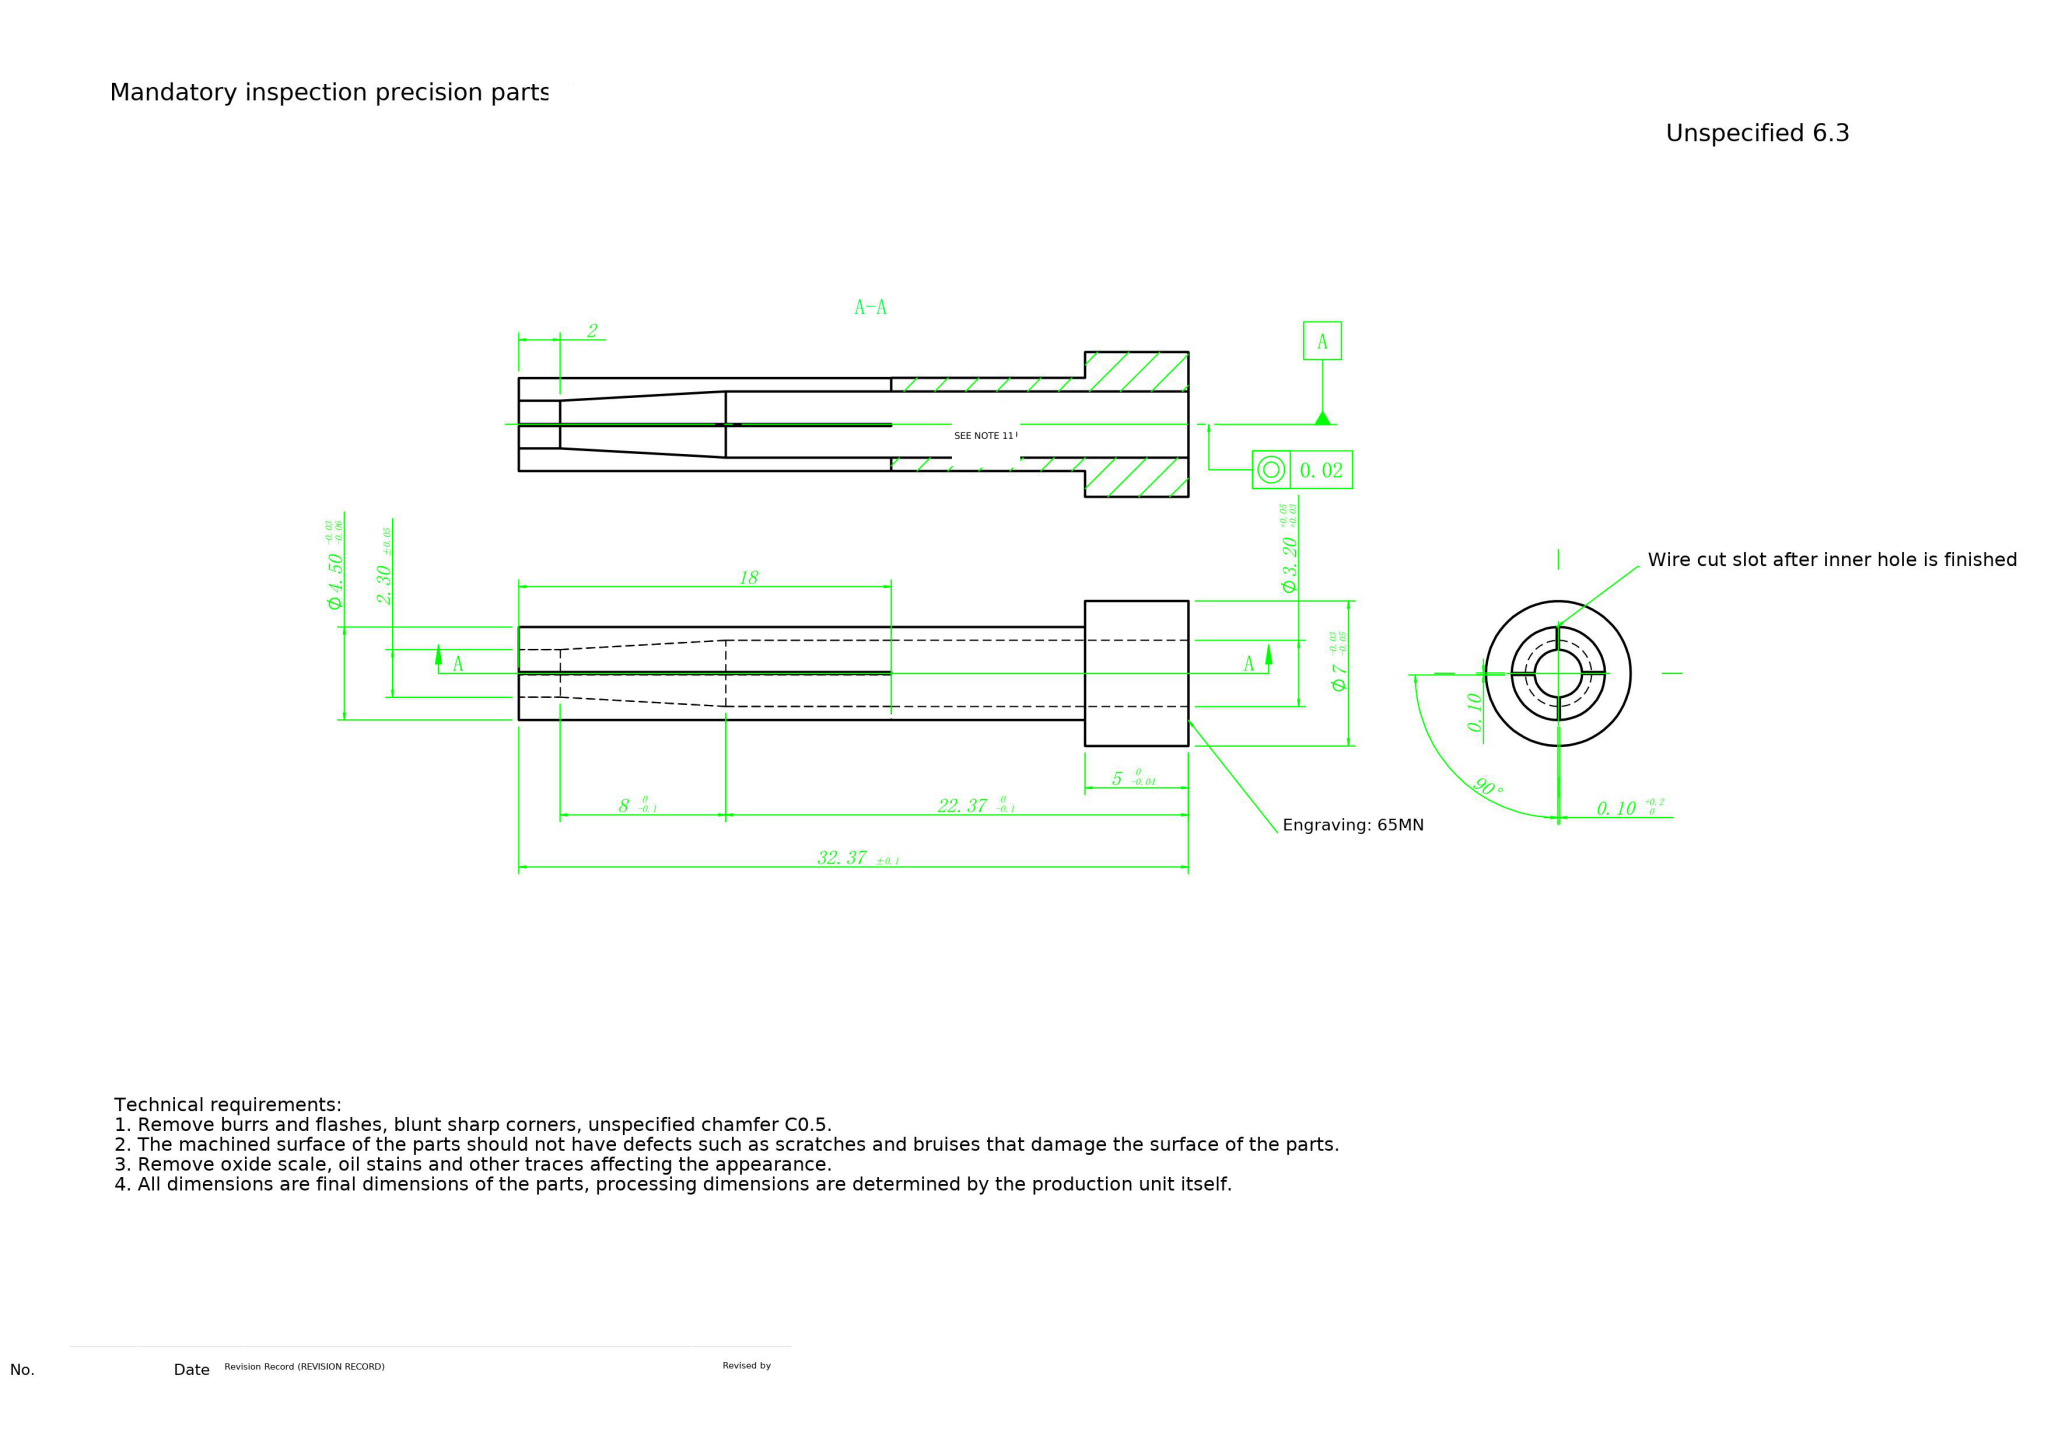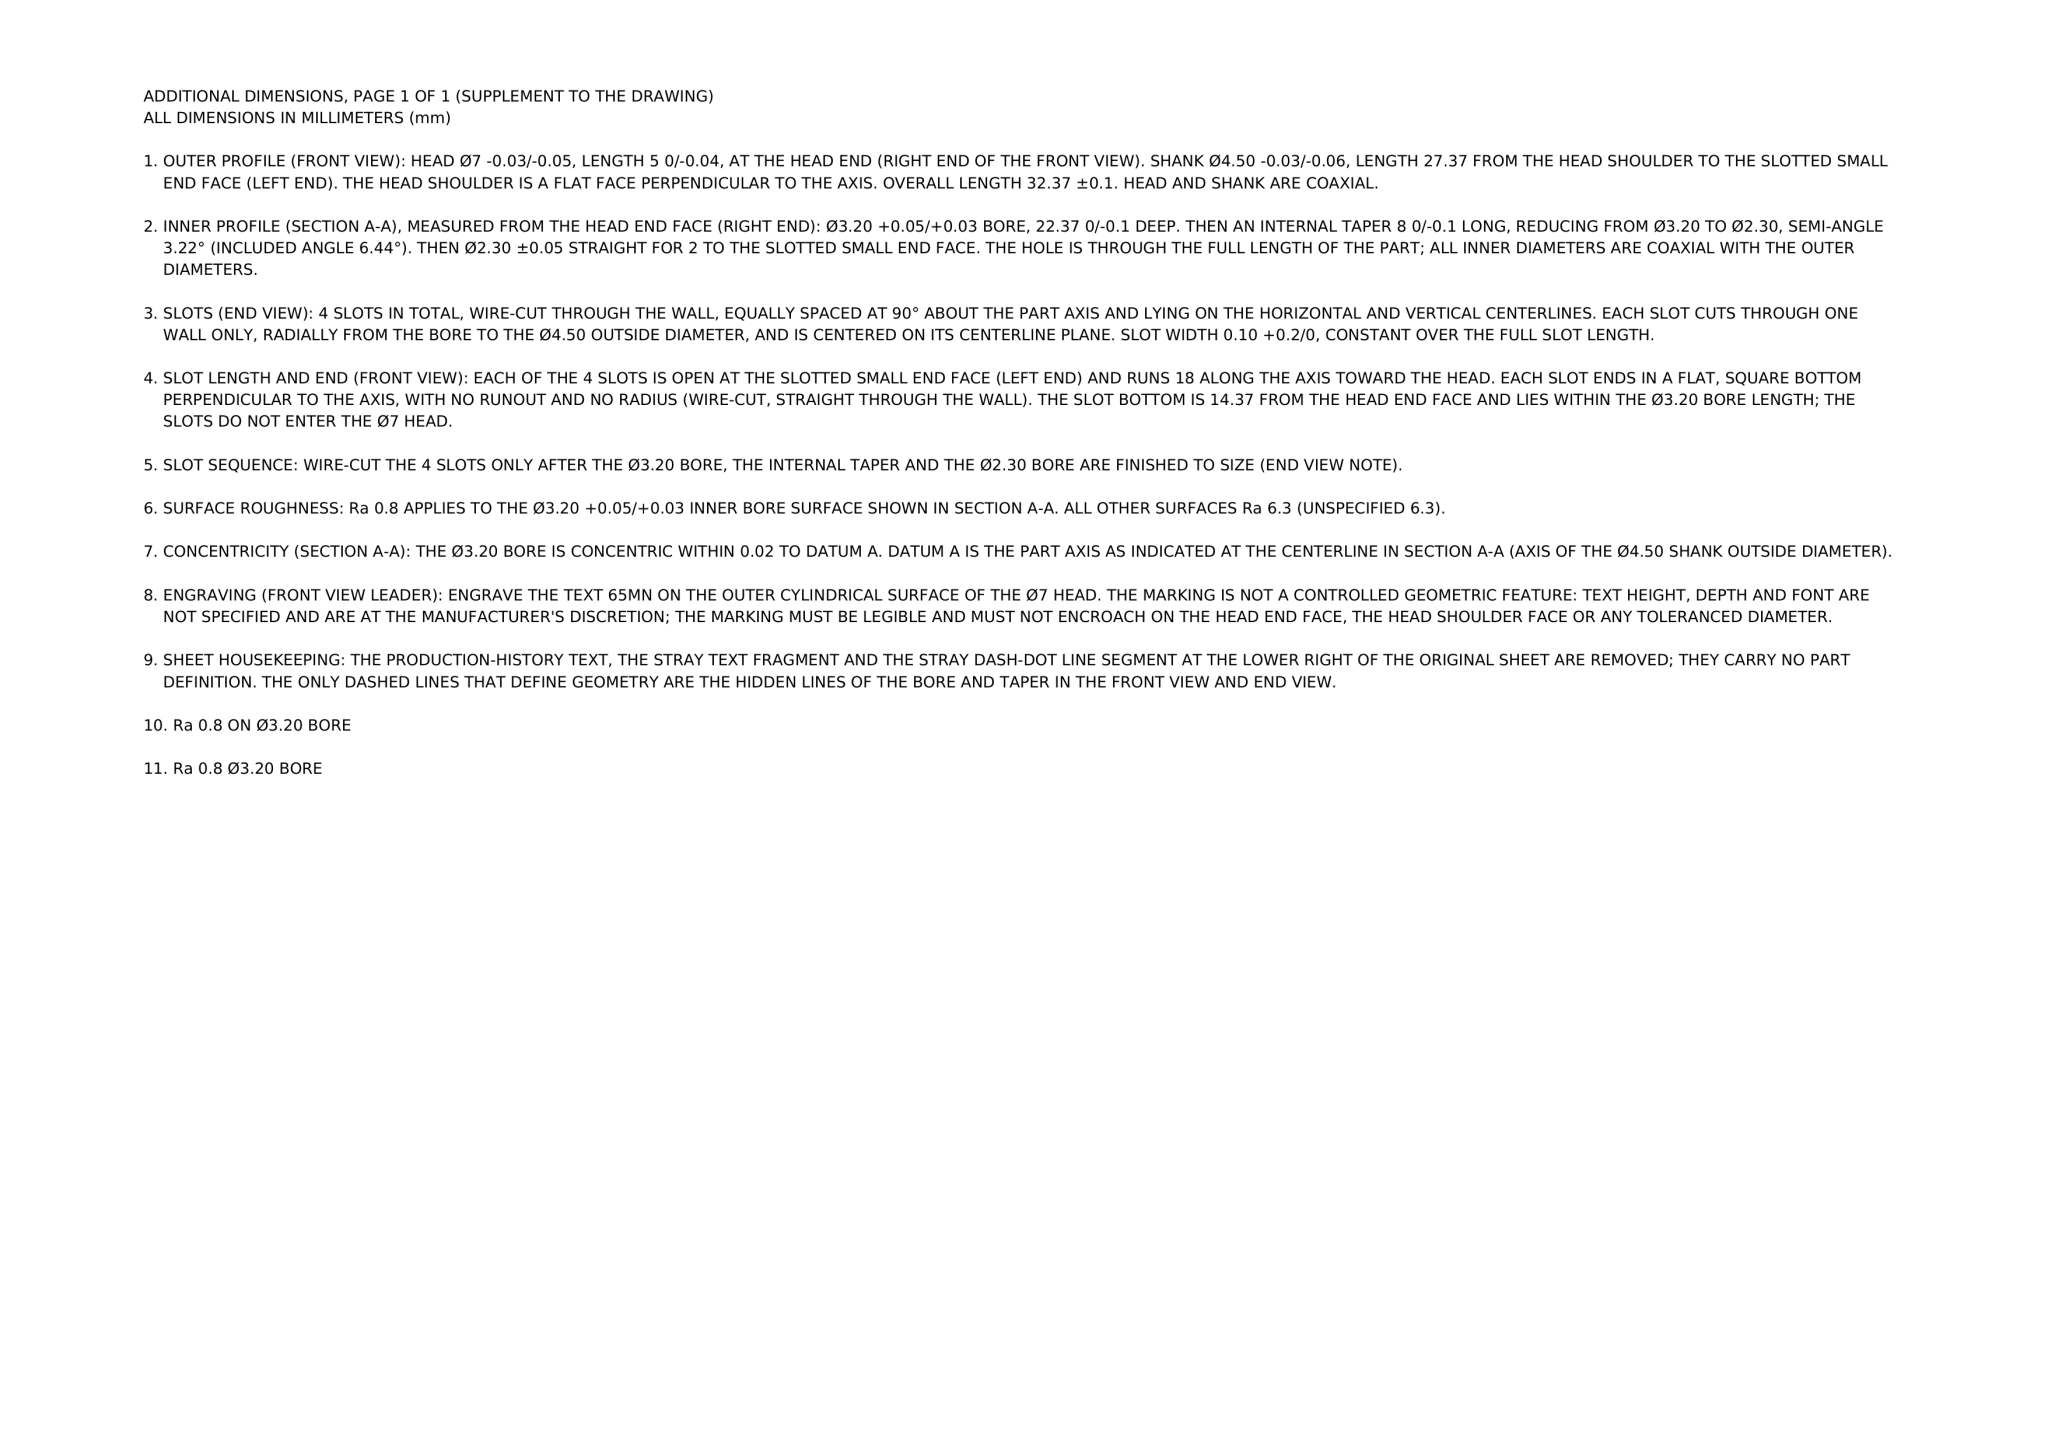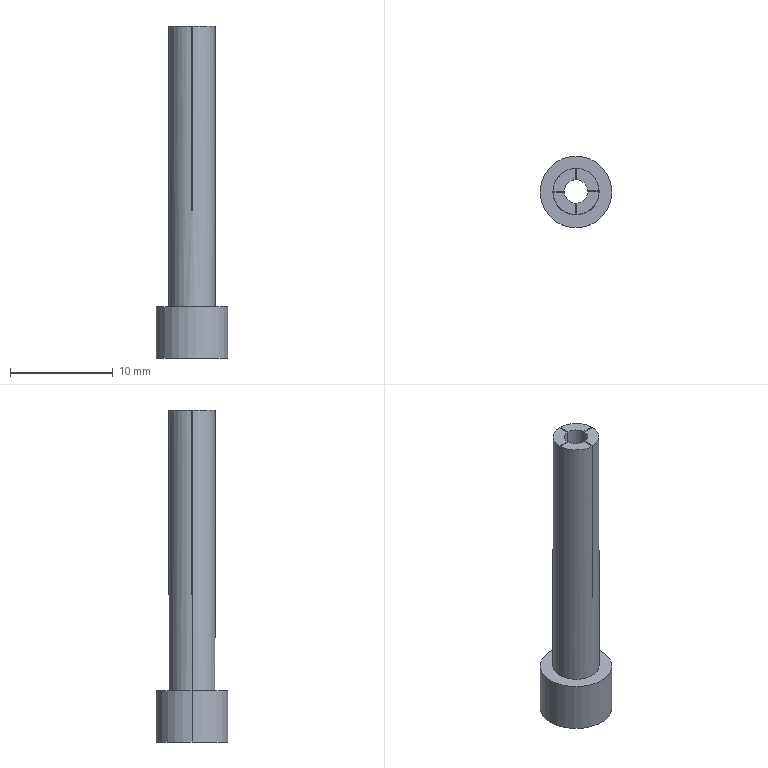Part | NX | mm | 1 solid | 32 faces | box 7 x 7 x 32.37 mm | volume 386 mm3 | plane 18 | cylinder 10 | cone 4 | commonest cylinder face diameters 2.3 x4 7 x2 3.2 x2 4.5 x2